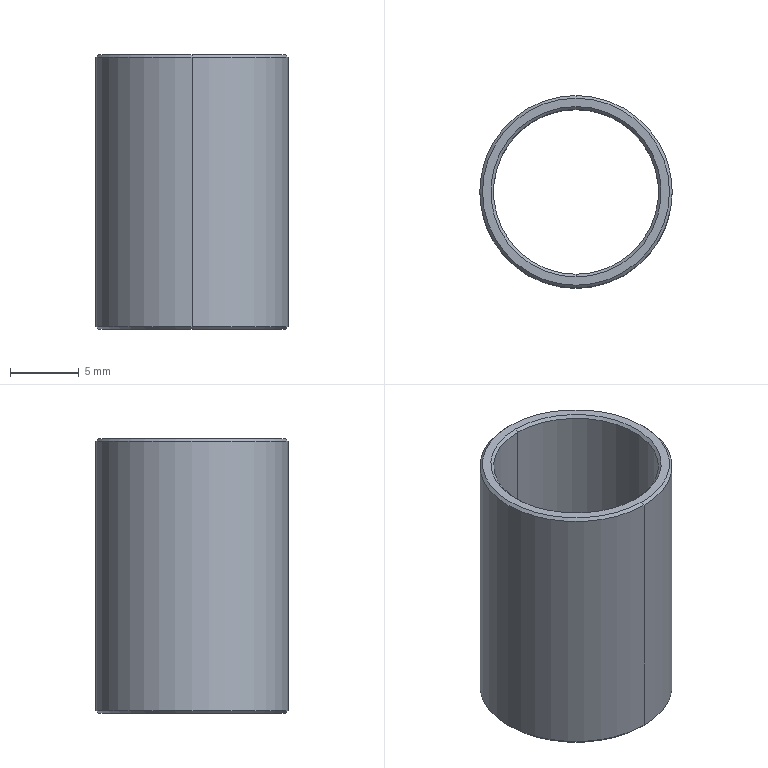Component | SolidWorks | 53-3 | 1 solid | 14 faces | box 14 x 14 x 20 mm | volume 814 mm3 | cone 8 | cylinder 4 | plane 2 | commonest cylinder face diameters 14 x2 12 x2
build123d program:
from build123d import *

# Parameters (mm, degrees)
SKETCH1_W     = 1
SKETCH1_H     = 20
CHAMFER1_SIZE = 0.2


with BuildPart() as part:
    # Sketch1 → Revolve1 (revolve)
    with BuildSketch(Plane.XY, mode=Mode.PRIVATE) as revolve1_sk:
        with Locations((6.5, -10)):
            Rectangle(SKETCH1_W, SKETCH1_H)
    revolve(revolve1_sk.sketch.rotate(Axis((0, 0, 0), (0, -1, 0)), 90), axis=Axis((0, 0, 0), (0, -1, 0)))

    # Chamfer1
    chamfer1_edges = [part.edges().sort_by_distance(p)[0] for p in [
        (0, 0, -6),
        (0, 0, -7),
        (0, -20, -7),
        (0, -20, -6),
    ]]
    chamfer(chamfer1_edges, length=CHAMFER1_SIZE)


solid = part.part

# Placed as in the assembly
solid = solid.moved(Location((0, -38, 51.394), (90, 0, 0)))
STEP:
#1=COLOUR_RGB('',0.7922,0.8196,0.9333);
#2=FILL_AREA_STYLE_COLOUR('',#1);
#3=FILL_AREA_STYLE('',(#2));
#4=SURFACE_STYLE_FILL_AREA(#3);
#5=SURFACE_SIDE_STYLE('',(#4));
#6=SURFACE_STYLE_USAGE(.BOTH.,#5);
#7=PRESENTATION_STYLE_ASSIGNMENT((#6));
#8=CARTESIAN_POINT('',(-0.,-1.228,1.236));
#9=VERTEX_POINT('',#8);
#10=CARTESIAN_POINT('',(-0.,-1.764,1.236));
#11=VERTEX_POINT('',#10);
#12=CARTESIAN_POINT('',(-0.,-1.496,1.236));
#13=DIRECTION('',(-0.,-0.,-1.));
#14=DIRECTION('',(0.,-1.,0.));
#15=AXIS2_PLACEMENT_3D('',#12,#13,#14);
#16=CIRCLE('',#15,0.2677);
#17=EDGE_CURVE('',#9,#11,#16,.T.);
#18=ORIENTED_EDGE('',*,*,#17,.F.);
#19=CARTESIAN_POINT('',(-0.,-1.22,1.244));
#20=VERTEX_POINT('',#19);
#21=CARTESIAN_POINT('',(-0.,-1.228,1.236));
#22=DIRECTION('',(0.,0.7071,0.7071));
#23=VECTOR('',#22,39.37);
#24=LINE('',#21,#23);
#25=EDGE_CURVE('',#9,#20,#24,.T.);
#26=ORIENTED_EDGE('',*,*,#25,.T.);
#27=CARTESIAN_POINT('',(-0.,-1.772,1.244));
#28=VERTEX_POINT('',#27);
#29=CARTESIAN_POINT('',(-0.,-1.496,1.244));
#30=DIRECTION('',(0.,0.,1.));
#31=DIRECTION('',(0.,-1.,0.));
#32=AXIS2_PLACEMENT_3D('',#29,#30,#31);
#33=CIRCLE('',#32,0.2756);
#34=EDGE_CURVE('',#28,#20,#33,.T.);
#35=ORIENTED_EDGE('',*,*,#34,.F.);
#36=CARTESIAN_POINT('',(-0.,-1.764,1.236));
#37=DIRECTION('',(0.,-0.7071,0.7071));
#38=VECTOR('',#37,39.37);
#39=LINE('',#36,#38);
#40=EDGE_CURVE('',#11,#28,#39,.T.);
#41=ORIENTED_EDGE('',*,*,#40,.F.);
#42=EDGE_LOOP('',(#18,#26,#35,#41));
#43=FACE_OUTER_BOUND('',#42,.T.);
#44=CARTESIAN_POINT('',(-0.,-1.496,1.236));
#45=DIRECTION('',(0.,0.,1.));
#46=DIRECTION('',(0.,-1.,0.));
#47=AXIS2_PLACEMENT_3D('',#44,#45,#46);
#48=CONICAL_SURFACE('',#47,0.2677,0.7854);
#49=ADVANCED_FACE('',(#43),#48,.T.);
#50=CARTESIAN_POINT('',(-0.,-1.732,1.244));
#51=VERTEX_POINT('',#50);
#52=CARTESIAN_POINT('',(-0.,-1.26,1.244));
#53=VERTEX_POINT('',#52);
#54=CARTESIAN_POINT('',(-0.,-1.496,1.244));
#55=DIRECTION('',(-0.,-0.,-1.));
#56=DIRECTION('',(0.,-1.,0.));
#57=AXIS2_PLACEMENT_3D('',#54,#55,#56);
#58=CIRCLE('',#57,0.2362);
#59=EDGE_CURVE('',#51,#53,#58,.T.);
#60=ORIENTED_EDGE('',*,*,#59,.F.);
#61=CARTESIAN_POINT('',(-0.,-1.74,1.236));
#62=VERTEX_POINT('',#61);
#63=CARTESIAN_POINT('',(-0.,-1.732,1.244));
#64=DIRECTION('',(0.,-0.7071,-0.7071));
#65=VECTOR('',#64,39.37);
#66=LINE('',#63,#65);
#67=EDGE_CURVE('',#51,#62,#66,.T.);
#68=ORIENTED_EDGE('',*,*,#67,.T.);
#69=CARTESIAN_POINT('',(-0.,-1.252,1.236));
#70=VERTEX_POINT('',#69);
#71=CARTESIAN_POINT('',(-0.,-1.496,1.236));
#72=DIRECTION('',(0.,0.,1.));
#73=DIRECTION('',(0.,-1.,0.));
#74=AXIS2_PLACEMENT_3D('',#71,#72,#73);
#75=CIRCLE('',#74,0.2441);
#76=EDGE_CURVE('',#70,#62,#75,.T.);
#77=ORIENTED_EDGE('',*,*,#76,.F.);
#78=CARTESIAN_POINT('',(-0.,-1.26,1.244));
#79=DIRECTION('',(-0.,0.7071,-0.7071));
#80=VECTOR('',#79,39.37);
#81=LINE('',#78,#80);
#82=EDGE_CURVE('',#53,#70,#81,.T.);
#83=ORIENTED_EDGE('',*,*,#82,.F.);
#84=EDGE_LOOP('',(#60,#68,#77,#83));
#85=FACE_OUTER_BOUND('',#84,.T.);
#86=CARTESIAN_POINT('',(-0.,-1.496,1.244));
#87=DIRECTION('',(-0.,-0.,-1.));
#88=DIRECTION('',(0.,1.,0.));
#89=AXIS2_PLACEMENT_3D('',#86,#87,#88);
#90=CONICAL_SURFACE('',#89,0.2362,0.7854);
#91=ADVANCED_FACE('',(#85),#90,.F.);
#92=CARTESIAN_POINT('',(-0.,-1.764,2.023));
#93=VERTEX_POINT('',#92);
#94=CARTESIAN_POINT('',(-0.,-1.228,2.023));
#95=VERTEX_POINT('',#94);
#96=CARTESIAN_POINT('',(-0.,-1.496,2.023));
#97=DIRECTION('',(0.,0.,1.));
#98=DIRECTION('',(0.,1.,0.));
#99=AXIS2_PLACEMENT_3D('',#96,#97,#98);
#100=CIRCLE('',#99,0.2677);
#101=EDGE_CURVE('',#93,#95,#100,.T.);
#102=ORIENTED_EDGE('',*,*,#101,.F.);
#103=CARTESIAN_POINT('',(-0.,-1.772,2.016));
#104=VERTEX_POINT('',#103);
#105=CARTESIAN_POINT('',(-0.,-1.772,2.016));
#106=DIRECTION('',(0.,-0.7071,-0.7071));
#107=VECTOR('',#106,39.37);
#108=LINE('',#105,#107);
#109=EDGE_CURVE('',#93,#104,#108,.T.);
#110=ORIENTED_EDGE('',*,*,#109,.T.);
#111=CARTESIAN_POINT('',(-0.,-1.22,2.016));
#112=VERTEX_POINT('',#111);
#113=CARTESIAN_POINT('',(-0.,-1.496,2.016));
#114=DIRECTION('',(-0.,-0.,-1.));
#115=DIRECTION('',(0.,1.,0.));
#116=AXIS2_PLACEMENT_3D('',#113,#114,#115);
#117=CIRCLE('',#116,0.2756);
#118=EDGE_CURVE('',#112,#104,#117,.T.);
#119=ORIENTED_EDGE('',*,*,#118,.F.);
#120=CARTESIAN_POINT('',(-0.,-1.22,2.016));
#121=DIRECTION('',(-0.,0.7071,-0.7071));
#122=VECTOR('',#121,39.37);
#123=LINE('',#120,#122);
#124=EDGE_CURVE('',#95,#112,#123,.T.);
#125=ORIENTED_EDGE('',*,*,#124,.F.);
#126=EDGE_LOOP('',(#102,#110,#119,#125));
#127=FACE_OUTER_BOUND('',#126,.T.);
#128=CARTESIAN_POINT('',(-0.,-1.496,2.016));
#129=DIRECTION('',(-0.,-0.,-1.));
#130=DIRECTION('',(0.,1.,0.));
#131=AXIS2_PLACEMENT_3D('',#128,#129,#130);
#132=CONICAL_SURFACE('',#131,0.2756,0.7854);
#133=ADVANCED_FACE('',(#127),#132,.T.);
#134=CARTESIAN_POINT('',(-0.,-1.26,2.016));
#135=VERTEX_POINT('',#134);
#136=CARTESIAN_POINT('',(-0.,-1.732,2.016));
#137=VERTEX_POINT('',#136);
#138=CARTESIAN_POINT('',(-0.,-1.496,2.016));
#139=DIRECTION('',(0.,0.,1.));
#140=DIRECTION('',(0.,1.,0.));
#141=AXIS2_PLACEMENT_3D('',#138,#139,#140);
#142=CIRCLE('',#141,0.2362);
#143=EDGE_CURVE('',#135,#137,#142,.T.);
#144=ORIENTED_EDGE('',*,*,#143,.F.);
#145=CARTESIAN_POINT('',(-0.,-1.252,2.023));
#146=VERTEX_POINT('',#145);
#147=CARTESIAN_POINT('',(-0.,-1.252,2.023));
#148=DIRECTION('',(0.,0.7071,0.7071));
#149=VECTOR('',#148,39.37);
#150=LINE('',#147,#149);
#151=EDGE_CURVE('',#135,#146,#150,.T.);
#152=ORIENTED_EDGE('',*,*,#151,.T.);
#153=CARTESIAN_POINT('',(-0.,-1.74,2.023));
#154=VERTEX_POINT('',#153);
#155=CARTESIAN_POINT('',(-0.,-1.496,2.023));
#156=DIRECTION('',(-0.,-0.,-1.));
#157=DIRECTION('',(0.,1.,0.));
#158=AXIS2_PLACEMENT_3D('',#155,#156,#157);
#159=CIRCLE('',#158,0.2441);
#160=EDGE_CURVE('',#154,#146,#159,.T.);
#161=ORIENTED_EDGE('',*,*,#160,.F.);
#162=CARTESIAN_POINT('',(-0.,-1.74,2.023));
#163=DIRECTION('',(0.,-0.7071,0.7071));
#164=VECTOR('',#163,39.37);
#165=LINE('',#162,#164);
#166=EDGE_CURVE('',#137,#154,#165,.T.);
#167=ORIENTED_EDGE('',*,*,#166,.F.);
#168=EDGE_LOOP('',(#144,#152,#161,#167));
#169=FACE_OUTER_BOUND('',#168,.T.);
#170=CARTESIAN_POINT('',(-0.,-1.496,2.023));
#171=DIRECTION('',(0.,0.,1.));
#172=DIRECTION('',(0.,-1.,0.));
#173=AXIS2_PLACEMENT_3D('',#170,#171,#172);
#174=CONICAL_SURFACE('',#173,0.2441,0.7854);
#175=ADVANCED_FACE('',(#169),#174,.F.);
#176=ORIENTED_EDGE('',*,*,#118,.T.);
#177=CARTESIAN_POINT('',(-0.,-1.772,1.236));
#178=DIRECTION('',(-0.,-0.,-1.));
#179=VECTOR('',#178,39.37);
#180=LINE('',#177,#179);
#181=EDGE_CURVE('',#104,#28,#180,.T.);
#182=ORIENTED_EDGE('',*,*,#181,.T.);
#183=ORIENTED_EDGE('',*,*,#34,.T.);
#184=CARTESIAN_POINT('',(-0.,-1.22,1.236));
#185=DIRECTION('',(-0.,-0.,-1.));
#186=VECTOR('',#185,39.37);
#187=LINE('',#184,#186);
#188=EDGE_CURVE('',#112,#20,#187,.T.);
#189=ORIENTED_EDGE('',*,*,#188,.F.);
#190=EDGE_LOOP('',(#176,#182,#183,#189));
#191=FACE_OUTER_BOUND('',#190,.T.);
#192=CARTESIAN_POINT('',(-0.,-1.496,1.236));
#193=DIRECTION('',(-0.,-0.,-1.));
#194=DIRECTION('',(0.,1.,0.));
#195=AXIS2_PLACEMENT_3D('',#192,#193,#194);
#196=CYLINDRICAL_SURFACE('',#195,0.2756);
#197=ADVANCED_FACE('',(#191),#196,.T.);
#198=ORIENTED_EDGE('',*,*,#143,.T.);
#199=CARTESIAN_POINT('',(-0.,-1.732,1.236));
#200=DIRECTION('',(-0.,-0.,-1.));
#201=VECTOR('',#200,39.37);
#202=LINE('',#199,#201);
#203=EDGE_CURVE('',#137,#51,#202,.T.);
#204=ORIENTED_EDGE('',*,*,#203,.T.);
#205=ORIENTED_EDGE('',*,*,#59,.T.);
#206=CARTESIAN_POINT('',(-0.,-1.26,1.236));
#207=DIRECTION('',(-0.,-0.,-1.));
#208=VECTOR('',#207,39.37);
#209=LINE('',#206,#208);
#210=EDGE_CURVE('',#135,#53,#209,.T.);
#211=ORIENTED_EDGE('',*,*,#210,.F.);
#212=EDGE_LOOP('',(#198,#204,#205,#211));
#213=FACE_OUTER_BOUND('',#212,.T.);
#214=CARTESIAN_POINT('',(-0.,-1.496,1.236));
#215=DIRECTION('',(-0.,-0.,-1.));
#216=DIRECTION('',(0.,1.,0.));
#217=AXIS2_PLACEMENT_3D('',#214,#215,#216);
#218=CYLINDRICAL_SURFACE('',#217,0.2362);
#219=ADVANCED_FACE('',(#213),#218,.F.);
#220=ORIENTED_EDGE('',*,*,#203,.F.);
#221=CARTESIAN_POINT('',(-0.,-1.496,2.016));
#222=DIRECTION('',(0.,0.,1.));
#223=DIRECTION('',(0.,1.,0.));
#224=AXIS2_PLACEMENT_3D('',#221,#222,#223);
#225=CIRCLE('',#224,0.2362);
#226=EDGE_CURVE('',#137,#135,#225,.T.);
#227=ORIENTED_EDGE('',*,*,#226,.T.);
#228=ORIENTED_EDGE('',*,*,#210,.T.);
#229=CARTESIAN_POINT('',(-0.,-1.496,1.244));
#230=DIRECTION('',(-0.,-0.,-1.));
#231=DIRECTION('',(0.,-1.,0.));
#232=AXIS2_PLACEMENT_3D('',#229,#230,#231);
#233=CIRCLE('',#232,0.2362);
#234=EDGE_CURVE('',#53,#51,#233,.T.);
#235=ORIENTED_EDGE('',*,*,#234,.T.);
#236=EDGE_LOOP('',(#220,#227,#228,#235));
#237=FACE_OUTER_BOUND('',#236,.T.);
#238=CARTESIAN_POINT('',(-0.,-1.496,1.236));
#239=DIRECTION('',(-0.,-0.,-1.));
#240=DIRECTION('',(0.,1.,0.));
#241=AXIS2_PLACEMENT_3D('',#238,#239,#240);
#242=CYLINDRICAL_SURFACE('',#241,0.2362);
#243=ADVANCED_FACE('',(#237),#242,.F.);
#244=ORIENTED_EDGE('',*,*,#160,.T.);
#245=CARTESIAN_POINT('',(-0.,-1.496,2.023));
#246=DIRECTION('',(-0.,-0.,-1.));
#247=DIRECTION('',(0.,1.,0.));
#248=AXIS2_PLACEMENT_3D('',#245,#246,#247);
#249=CIRCLE('',#248,0.2441);
#250=EDGE_CURVE('',#146,#154,#249,.T.);
#251=ORIENTED_EDGE('',*,*,#250,.T.);
#252=EDGE_LOOP('',(#244,#251));
#253=FACE_BOUND('',#252,.T.);
#254=CARTESIAN_POINT('',(-0.,-1.496,2.023));
#255=DIRECTION('',(0.,0.,1.));
#256=DIRECTION('',(0.,1.,0.));
#257=AXIS2_PLACEMENT_3D('',#254,#255,#256);
#258=CIRCLE('',#257,0.2677);
#259=EDGE_CURVE('',#95,#93,#258,.T.);
#260=ORIENTED_EDGE('',*,*,#259,.T.);
#261=ORIENTED_EDGE('',*,*,#101,.T.);
#262=EDGE_LOOP('',(#260,#261));
#263=FACE_OUTER_BOUND('',#262,.T.);
#264=CARTESIAN_POINT('',(0.2362,-1.496,2.023));
#265=DIRECTION('',(-0.,-0.,-1.));
#266=DIRECTION('',(-0.,1.,-0.));
#267=AXIS2_PLACEMENT_3D('',#264,#265,#266);
#268=PLANE('',#267);
#269=ADVANCED_FACE('',(#253,#263),#268,.F.);
#270=ORIENTED_EDGE('',*,*,#181,.F.);
#271=CARTESIAN_POINT('',(-0.,-1.496,2.016));
#272=DIRECTION('',(-0.,-0.,-1.));
#273=DIRECTION('',(0.,1.,0.));
#274=AXIS2_PLACEMENT_3D('',#271,#272,#273);
#275=CIRCLE('',#274,0.2756);
#276=EDGE_CURVE('',#104,#112,#275,.T.);
#277=ORIENTED_EDGE('',*,*,#276,.T.);
#278=ORIENTED_EDGE('',*,*,#188,.T.);
#279=CARTESIAN_POINT('',(-0.,-1.496,1.244));
#280=DIRECTION('',(0.,0.,1.));
#281=DIRECTION('',(0.,-1.,0.));
#282=AXIS2_PLACEMENT_3D('',#279,#280,#281);
#283=CIRCLE('',#282,0.2756);
#284=EDGE_CURVE('',#20,#28,#283,.T.);
#285=ORIENTED_EDGE('',*,*,#284,.T.);
#286=EDGE_LOOP('',(#270,#277,#278,#285));
#287=FACE_OUTER_BOUND('',#286,.T.);
#288=CARTESIAN_POINT('',(-0.,-1.496,1.236));
#289=DIRECTION('',(-0.,-0.,-1.));
#290=DIRECTION('',(0.,1.,0.));
#291=AXIS2_PLACEMENT_3D('',#288,#289,#290);
#292=CYLINDRICAL_SURFACE('',#291,0.2756);
#293=ADVANCED_FACE('',(#287),#292,.T.);
#294=ORIENTED_EDGE('',*,*,#76,.T.);
#295=CARTESIAN_POINT('',(-0.,-1.496,1.236));
#296=DIRECTION('',(0.,0.,1.));
#297=DIRECTION('',(0.,-1.,0.));
#298=AXIS2_PLACEMENT_3D('',#295,#296,#297);
#299=CIRCLE('',#298,0.2441);
#300=EDGE_CURVE('',#62,#70,#299,.T.);
#301=ORIENTED_EDGE('',*,*,#300,.T.);
#302=EDGE_LOOP('',(#294,#301));
#303=FACE_BOUND('',#302,.T.);
#304=CARTESIAN_POINT('',(-0.,-1.496,1.236));
#305=DIRECTION('',(-0.,-0.,-1.));
#306=DIRECTION('',(0.,-1.,0.));
#307=AXIS2_PLACEMENT_3D('',#304,#305,#306);
#308=CIRCLE('',#307,0.2677);
#309=EDGE_CURVE('',#11,#9,#308,.T.);
#310=ORIENTED_EDGE('',*,*,#309,.T.);
#311=ORIENTED_EDGE('',*,*,#17,.T.);
#312=EDGE_LOOP('',(#310,#311));
#313=FACE_OUTER_BOUND('',#312,.T.);
#314=CARTESIAN_POINT('',(0.2362,-1.496,1.236));
#315=DIRECTION('',(0.,0.,1.));
#316=DIRECTION('',(0.,-1.,0.));
#317=AXIS2_PLACEMENT_3D('',#314,#315,#316);
#318=PLANE('',#317);
#319=ADVANCED_FACE('',(#303,#313),#318,.F.);
#320=ORIENTED_EDGE('',*,*,#151,.F.);
#321=ORIENTED_EDGE('',*,*,#226,.F.);
#322=ORIENTED_EDGE('',*,*,#166,.T.);
#323=ORIENTED_EDGE('',*,*,#250,.F.);
#324=EDGE_LOOP('',(#320,#321,#322,#323));
#325=FACE_OUTER_BOUND('',#324,.T.);
#326=CARTESIAN_POINT('',(-0.,-1.496,2.023));
#327=DIRECTION('',(0.,0.,1.));
#328=DIRECTION('',(0.,-1.,0.));
#329=AXIS2_PLACEMENT_3D('',#326,#327,#328);
#330=CONICAL_SURFACE('',#329,0.2441,0.7854);
#331=ADVANCED_FACE('',(#325),#330,.F.);
#332=ORIENTED_EDGE('',*,*,#109,.F.);
#333=ORIENTED_EDGE('',*,*,#259,.F.);
#334=ORIENTED_EDGE('',*,*,#124,.T.);
#335=ORIENTED_EDGE('',*,*,#276,.F.);
#336=EDGE_LOOP('',(#332,#333,#334,#335));
#337=FACE_OUTER_BOUND('',#336,.T.);
#338=CARTESIAN_POINT('',(-0.,-1.496,2.016));
#339=DIRECTION('',(-0.,-0.,-1.));
#340=DIRECTION('',(0.,1.,0.));
#341=AXIS2_PLACEMENT_3D('',#338,#339,#340);
#342=CONICAL_SURFACE('',#341,0.2756,0.7854);
#343=ADVANCED_FACE('',(#337),#342,.T.);
#344=ORIENTED_EDGE('',*,*,#67,.F.);
#345=ORIENTED_EDGE('',*,*,#234,.F.);
#346=ORIENTED_EDGE('',*,*,#82,.T.);
#347=ORIENTED_EDGE('',*,*,#300,.F.);
#348=EDGE_LOOP('',(#344,#345,#346,#347));
#349=FACE_OUTER_BOUND('',#348,.T.);
#350=CARTESIAN_POINT('',(-0.,-1.496,1.244));
#351=DIRECTION('',(-0.,-0.,-1.));
#352=DIRECTION('',(0.,1.,0.));
#353=AXIS2_PLACEMENT_3D('',#350,#351,#352);
#354=CONICAL_SURFACE('',#353,0.2362,0.7854);
#355=ADVANCED_FACE('',(#349),#354,.F.);
#356=ORIENTED_EDGE('',*,*,#25,.F.);
#357=ORIENTED_EDGE('',*,*,#309,.F.);
#358=ORIENTED_EDGE('',*,*,#40,.T.);
#359=ORIENTED_EDGE('',*,*,#284,.F.);
#360=EDGE_LOOP('',(#356,#357,#358,#359));
#361=FACE_OUTER_BOUND('',#360,.T.);
#362=CARTESIAN_POINT('',(-0.,-1.496,1.236));
#363=DIRECTION('',(0.,0.,1.));
#364=DIRECTION('',(0.,-1.,0.));
#365=AXIS2_PLACEMENT_3D('',#362,#363,#364);
#366=CONICAL_SURFACE('',#365,0.2677,0.7854);
#367=ADVANCED_FACE('',(#361),#366,.T.);
#368=CLOSED_SHELL('',(#49,#91,#133,#175,#197,#219,#243,#269,#293,#319,#331,#343,#355,#367));
#369=MANIFOLD_SOLID_BREP('',#368);
#370=STYLED_ITEM('',(#7),#369);
#371=PRESENTATION_LAYER_ASSIGNMENT('','',(#370));
#372=CARTESIAN_POINT('',(0.,0.,0.));
#373=DIRECTION('',(0.,0.,1.));
#374=DIRECTION('',(1.,0.,0.));
#375=AXIS2_PLACEMENT_3D('',#372,#373,#374);
#376=(LENGTH_UNIT()NAMED_UNIT(*)SI_UNIT($,.METRE.));
#377=LENGTH_MEASURE_WITH_UNIT(LENGTH_MEASURE(0.0254),#376);
#378=DIMENSIONAL_EXPONENTS(1.,0.,0.,0.,0.,0.,0.);
#379=(CONVERSION_BASED_UNIT('',#377)LENGTH_UNIT()NAMED_UNIT(#378));
#380=UNCERTAINTY_MEASURE_WITH_UNIT(LENGTH_MEASURE(0.00001),#379,'','');
#381=(NAMED_UNIT(*)PLANE_ANGLE_UNIT()SI_UNIT($,.RADIAN.));
#382=(NAMED_UNIT(*)SI_UNIT($,.STERADIAN.)SOLID_ANGLE_UNIT());
#383=(GEOMETRIC_REPRESENTATION_CONTEXT(3)GLOBAL_UNCERTAINTY_ASSIGNED_CONTEXT((#380))GLOBAL_UNIT_ASSIGNED_CONTEXT((#379,#381,#382))REPRESENTATION_CONTEXT('',''));
#384=ADVANCED_BREP_SHAPE_REPRESENTATION('',(#369,#375),#383);
#385=(LENGTH_UNIT()NAMED_UNIT(*)SI_UNIT($,.METRE.));
#386=LENGTH_MEASURE_WITH_UNIT(LENGTH_MEASURE(0.0254),#385);
#387=DIMENSIONAL_EXPONENTS(1.,0.,0.,0.,0.,0.,0.);
#388=(CONVERSION_BASED_UNIT('',#386)LENGTH_UNIT()NAMED_UNIT(#387));
#389=UNCERTAINTY_MEASURE_WITH_UNIT(LENGTH_MEASURE(0.00001),#388,'','');
#390=(NAMED_UNIT(*)PLANE_ANGLE_UNIT()SI_UNIT($,.RADIAN.));
#391=(NAMED_UNIT(*)SI_UNIT($,.STERADIAN.)SOLID_ANGLE_UNIT());
#392=(GEOMETRIC_REPRESENTATION_CONTEXT(3)GLOBAL_UNCERTAINTY_ASSIGNED_CONTEXT((#389))GLOBAL_UNIT_ASSIGNED_CONTEXT((#388,#390,#391))REPRESENTATION_CONTEXT('',''));
#393=MECHANICAL_DESIGN_GEOMETRIC_PRESENTATION_REPRESENTATION('',(#370),#392);